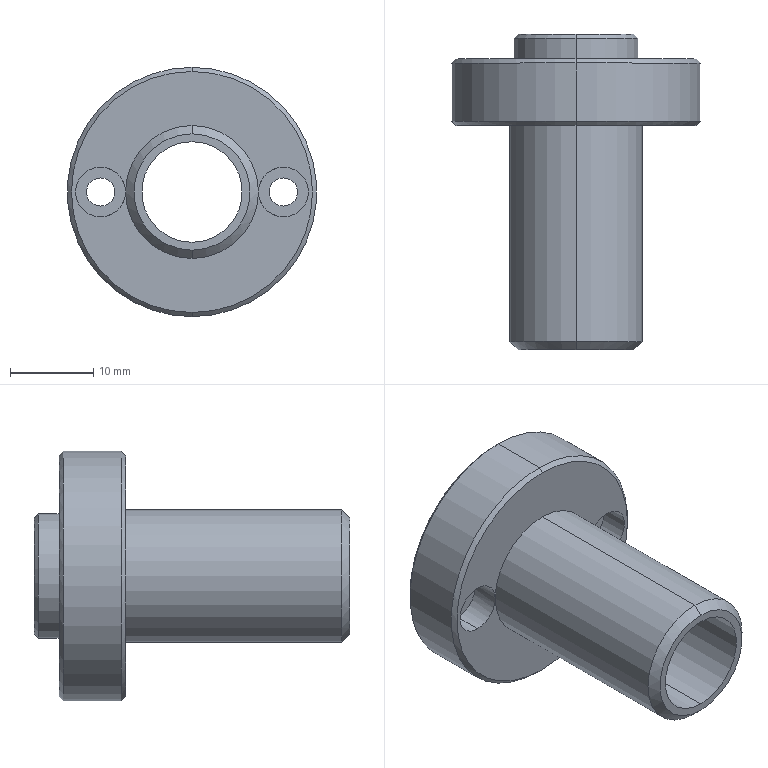Component | SolidWorks | GbgbLowerMagnetGuideTubeF8-1 | 1 solid | 30 faces | box 30 x 38 x 30 mm | volume 6915 mm3 | cylinder 16 | cone 8 | plane 6 | commonest cylinder face diameters 6 x4 3.4 x4 15 x2 30 x2 16 x2 12.1 x2
build123d program:
from build123d import *

# Parameters (mm, degrees)
CHAMFER1_SIZE                                        = 1
HOLE_SIZE_ACCORDING_TO_THE_TYPE_OF_HEX_S_D           = 3.4
HOLE_SIZE_ACCORDING_TO_THE_TYPE_OF_HEX_S_CBORE_D     = 6
HOLE_SIZE_ACCORDING_TO_THE_TYPE_OF_HEX_S_CBORE_DEPTH = 3.4
CHAMFER2_SIZE                                        = 0.5


with BuildPart() as part:
    # Sketch1 → Revolve1 (revolve)
    with BuildSketch(Plane.XY, mode=Mode.PRIVATE) as revolve1_sk:
        Polygon((-6.05, 38), (-6.05, 0), (-8, 0), (-8, 27), (-15, 27), (-15, 35), (-7.5, 35), (-7.5, 38), align=None)
    revolve(revolve1_sk.sketch.rotate(Axis((0, 48.525, 0), (0, -1, 0)), 270), axis=Axis((0, 48.525, 0), (0, -1, 0)))

    # Chamfer1
    chamfer1_edges = [part.edges().sort_by_distance(p)[0] for p in [
        (0, 0, -8),
    ]]
    chamfer(chamfer1_edges, length=CHAMFER1_SIZE)

    # Hole Size according to the type of hex s (through all)
    with Locations(Plane(origin=(0, 27, 0), x_dir=(-1, 0, 0), z_dir=(0, -1, 0))):
        with Locations((11, 0), (-11, 0)):
            CounterBoreHole(HOLE_SIZE_ACCORDING_TO_THE_TYPE_OF_HEX_S_D / 2, HOLE_SIZE_ACCORDING_TO_THE_TYPE_OF_HEX_S_CBORE_D / 2, HOLE_SIZE_ACCORDING_TO_THE_TYPE_OF_HEX_S_CBORE_DEPTH)

    # Chamfer2
    chamfer2_edges = [part.edges().sort_by_distance(p)[0] for p in [
        (0, 38, -7.5),
        (0, 35, -15),
        (0, 27, -15),
    ]]
    chamfer(chamfer2_edges, length=CHAMFER2_SIZE)


solid = part.part

# Placed as in the assembly
solid = solid.moved(Location((80.446, 337.44, 430.232), (0, 0, 0)))
STEP:
#1=CARTESIAN_POINT('',(3.167,14.781,17.214));
#2=VERTEX_POINT('',#1);
#3=CARTESIAN_POINT('',(3.167,14.781,16.663));
#4=VERTEX_POINT('',#3);
#5=CARTESIAN_POINT('',(3.167,14.781,16.938));
#6=DIRECTION('',(0.,1.,0.));
#7=DIRECTION('',(0.,0.,1.));
#8=AXIS2_PLACEMENT_3D('',#5,#6,#7);
#9=CIRCLE('',#8,0.2756);
#10=EDGE_CURVE('',#2,#4,#9,.T.);
#11=ORIENTED_EDGE('',*,*,#10,.F.);
#12=CARTESIAN_POINT('',(3.167,14.761,17.234));
#13=VERTEX_POINT('',#12);
#14=CARTESIAN_POINT('',(3.167,14.781,17.214));
#15=DIRECTION('',(0.,-0.7071,0.7071));
#16=VECTOR('',#15,39.37);
#17=LINE('',#14,#16);
#18=EDGE_CURVE('',#2,#13,#17,.T.);
#19=ORIENTED_EDGE('',*,*,#18,.T.);
#20=CARTESIAN_POINT('',(3.167,14.761,16.643));
#21=VERTEX_POINT('',#20);
#22=CARTESIAN_POINT('',(3.167,14.761,16.938));
#23=DIRECTION('',(0.,-1.,0.));
#24=DIRECTION('',(0.,0.,1.));
#25=AXIS2_PLACEMENT_3D('',#22,#23,#24);
#26=CIRCLE('',#25,0.2953);
#27=EDGE_CURVE('',#21,#13,#26,.T.);
#28=ORIENTED_EDGE('',*,*,#27,.F.);
#29=CARTESIAN_POINT('',(3.167,14.781,16.663));
#30=DIRECTION('',(0.,-0.7071,-0.7071));
#31=VECTOR('',#30,39.37);
#32=LINE('',#29,#31);
#33=EDGE_CURVE('',#4,#21,#32,.T.);
#34=ORIENTED_EDGE('',*,*,#33,.F.);
#35=EDGE_LOOP('',(#11,#19,#28,#34));
#36=FACE_OUTER_BOUND('',#35,.T.);
#37=CARTESIAN_POINT('',(3.167,14.781,16.938));
#38=DIRECTION('',(0.,-1.,0.));
#39=DIRECTION('',(0.,0.,-1.));
#40=AXIS2_PLACEMENT_3D('',#37,#38,#39);
#41=CONICAL_SURFACE('',#40,0.2756,0.7854);
#42=ADVANCED_FACE('',(#36),#41,.T.);
#43=CARTESIAN_POINT('',(3.167,14.348,16.367));
#44=VERTEX_POINT('',#43);
#45=CARTESIAN_POINT('',(3.167,14.348,17.509));
#46=VERTEX_POINT('',#45);
#47=CARTESIAN_POINT('',(3.167,14.348,16.938));
#48=DIRECTION('',(0.,-1.,0.));
#49=DIRECTION('',(0.,0.,-1.));
#50=AXIS2_PLACEMENT_3D('',#47,#48,#49);
#51=CIRCLE('',#50,0.5709);
#52=EDGE_CURVE('',#44,#46,#51,.T.);
#53=ORIENTED_EDGE('',*,*,#52,.F.);
#54=CARTESIAN_POINT('',(3.167,14.368,16.348));
#55=VERTEX_POINT('',#54);
#56=CARTESIAN_POINT('',(3.167,14.368,16.348));
#57=DIRECTION('',(0.,0.7071,-0.7071));
#58=VECTOR('',#57,39.37);
#59=LINE('',#56,#58);
#60=EDGE_CURVE('',#44,#55,#59,.T.);
#61=ORIENTED_EDGE('',*,*,#60,.T.);
#62=CARTESIAN_POINT('',(3.167,14.368,17.529));
#63=VERTEX_POINT('',#62);
#64=CARTESIAN_POINT('',(3.167,14.368,16.938));
#65=DIRECTION('',(0.,1.,0.));
#66=DIRECTION('',(0.,0.,-1.));
#67=AXIS2_PLACEMENT_3D('',#64,#65,#66);
#68=CIRCLE('',#67,0.5906);
#69=EDGE_CURVE('',#63,#55,#68,.T.);
#70=ORIENTED_EDGE('',*,*,#69,.F.);
#71=CARTESIAN_POINT('',(3.167,14.368,17.529));
#72=DIRECTION('',(0.,0.7071,0.7071));
#73=VECTOR('',#72,39.37);
#74=LINE('',#71,#73);
#75=EDGE_CURVE('',#46,#63,#74,.T.);
#76=ORIENTED_EDGE('',*,*,#75,.F.);
#77=EDGE_LOOP('',(#53,#61,#70,#76));
#78=FACE_OUTER_BOUND('',#77,.T.);
#79=CARTESIAN_POINT('',(3.167,14.368,16.938));
#80=DIRECTION('',(0.,1.,0.));
#81=DIRECTION('',(0.,0.,1.));
#82=AXIS2_PLACEMENT_3D('',#79,#80,#81);
#83=CONICAL_SURFACE('',#82,0.5906,0.7854);
#84=ADVANCED_FACE('',(#78),#83,.T.);
#85=CARTESIAN_POINT('',(3.167,14.663,17.509));
#86=VERTEX_POINT('',#85);
#87=CARTESIAN_POINT('',(3.167,14.663,16.367));
#88=VERTEX_POINT('',#87);
#89=CARTESIAN_POINT('',(3.167,14.663,16.938));
#90=DIRECTION('',(0.,1.,0.));
#91=DIRECTION('',(0.,0.,1.));
#92=AXIS2_PLACEMENT_3D('',#89,#90,#91);
#93=CIRCLE('',#92,0.5709);
#94=EDGE_CURVE('',#86,#88,#93,.T.);
#95=ORIENTED_EDGE('',*,*,#94,.F.);
#96=CARTESIAN_POINT('',(3.167,14.643,17.529));
#97=VERTEX_POINT('',#96);
#98=CARTESIAN_POINT('',(3.167,14.663,17.509));
#99=DIRECTION('',(0.,-0.7071,0.7071));
#100=VECTOR('',#99,39.37);
#101=LINE('',#98,#100);
#102=EDGE_CURVE('',#86,#97,#101,.T.);
#103=ORIENTED_EDGE('',*,*,#102,.T.);
#104=CARTESIAN_POINT('',(3.167,14.643,16.348));
#105=VERTEX_POINT('',#104);
#106=CARTESIAN_POINT('',(3.167,14.643,16.938));
#107=DIRECTION('',(0.,-1.,0.));
#108=DIRECTION('',(0.,0.,1.));
#109=AXIS2_PLACEMENT_3D('',#106,#107,#108);
#110=CIRCLE('',#109,0.5906);
#111=EDGE_CURVE('',#105,#97,#110,.T.);
#112=ORIENTED_EDGE('',*,*,#111,.F.);
#113=CARTESIAN_POINT('',(3.167,14.663,16.367));
#114=DIRECTION('',(0.,-0.7071,-0.7071));
#115=VECTOR('',#114,39.37);
#116=LINE('',#113,#115);
#117=EDGE_CURVE('',#88,#105,#116,.T.);
#118=ORIENTED_EDGE('',*,*,#117,.F.);
#119=EDGE_LOOP('',(#95,#103,#112,#118));
#120=FACE_OUTER_BOUND('',#119,.T.);
#121=CARTESIAN_POINT('',(3.167,14.663,16.938));
#122=DIRECTION('',(0.,-1.,0.));
#123=DIRECTION('',(0.,0.,-1.));
#124=AXIS2_PLACEMENT_3D('',#121,#122,#123);
#125=CONICAL_SURFACE('',#124,0.5709,0.7854);
#126=ADVANCED_FACE('',(#120),#125,.T.);
#127=CARTESIAN_POINT('',(2.734,14.482,17.056));
#128=VERTEX_POINT('',#127);
#129=CARTESIAN_POINT('',(2.734,14.482,16.82));
#130=VERTEX_POINT('',#129);
#131=CARTESIAN_POINT('',(2.734,14.482,16.938));
#132=DIRECTION('',(0.,-1.,0.));
#133=DIRECTION('',(0.,0.,-1.));
#134=AXIS2_PLACEMENT_3D('',#131,#132,#133);
#135=CIRCLE('',#134,0.1181);
#136=EDGE_CURVE('',#128,#130,#135,.T.);
#137=ORIENTED_EDGE('',*,*,#136,.F.);
#138=CARTESIAN_POINT('',(2.734,14.348,17.056));
#139=VERTEX_POINT('',#138);
#140=CARTESIAN_POINT('',(2.734,14.348,17.056));
#141=DIRECTION('',(0.,-1.,0.));
#142=VECTOR('',#141,39.37);
#143=LINE('',#140,#142);
#144=EDGE_CURVE('',#128,#139,#143,.T.);
#145=ORIENTED_EDGE('',*,*,#144,.T.);
#146=CARTESIAN_POINT('',(2.734,14.348,16.82));
#147=VERTEX_POINT('',#146);
#148=CARTESIAN_POINT('',(2.734,14.348,16.938));
#149=DIRECTION('',(0.,-1.,0.));
#150=DIRECTION('',(0.,0.,-1.));
#151=AXIS2_PLACEMENT_3D('',#148,#149,#150);
#152=CIRCLE('',#151,0.1181);
#153=EDGE_CURVE('',#139,#147,#152,.T.);
#154=ORIENTED_EDGE('',*,*,#153,.T.);
#155=CARTESIAN_POINT('',(2.734,14.348,16.82));
#156=DIRECTION('',(0.,-1.,0.));
#157=VECTOR('',#156,39.37);
#158=LINE('',#155,#157);
#159=EDGE_CURVE('',#130,#147,#158,.T.);
#160=ORIENTED_EDGE('',*,*,#159,.F.);
#161=EDGE_LOOP('',(#137,#145,#154,#160));
#162=FACE_OUTER_BOUND('',#161,.T.);
#163=CARTESIAN_POINT('',(2.734,14.348,16.938));
#164=DIRECTION('',(0.,-1.,0.));
#165=DIRECTION('',(0.,0.,-1.));
#166=AXIS2_PLACEMENT_3D('',#163,#164,#165);
#167=CYLINDRICAL_SURFACE('',#166,0.1181);
#168=ADVANCED_FACE('',(#162),#167,.F.);
#169=CARTESIAN_POINT('',(2.734,14.663,16.871));
#170=VERTEX_POINT('',#169);
#171=CARTESIAN_POINT('',(2.734,14.663,17.005));
#172=VERTEX_POINT('',#171);
#173=CARTESIAN_POINT('',(2.734,14.663,16.938));
#174=DIRECTION('',(0.,1.,0.));
#175=DIRECTION('',(0.,0.,1.));
#176=AXIS2_PLACEMENT_3D('',#173,#174,#175);
#177=CIRCLE('',#176,0.06693);
#178=EDGE_CURVE('',#170,#172,#177,.T.);
#179=ORIENTED_EDGE('',*,*,#178,.T.);
#180=CARTESIAN_POINT('',(2.734,14.482,17.005));
#181=VERTEX_POINT('',#180);
#182=CARTESIAN_POINT('',(2.734,14.348,17.005));
#183=DIRECTION('',(0.,-1.,0.));
#184=VECTOR('',#183,39.37);
#185=LINE('',#182,#184);
#186=EDGE_CURVE('',#172,#181,#185,.T.);
#187=ORIENTED_EDGE('',*,*,#186,.T.);
#188=CARTESIAN_POINT('',(2.734,14.482,16.871));
#189=VERTEX_POINT('',#188);
#190=CARTESIAN_POINT('',(2.734,14.482,16.938));
#191=DIRECTION('',(0.,-1.,0.));
#192=DIRECTION('',(0.,0.,-1.));
#193=AXIS2_PLACEMENT_3D('',#190,#191,#192);
#194=CIRCLE('',#193,0.06693);
#195=EDGE_CURVE('',#181,#189,#194,.T.);
#196=ORIENTED_EDGE('',*,*,#195,.T.);
#197=CARTESIAN_POINT('',(2.734,14.348,16.871));
#198=DIRECTION('',(0.,-1.,0.));
#199=VECTOR('',#198,39.37);
#200=LINE('',#197,#199);
#201=EDGE_CURVE('',#170,#189,#200,.T.);
#202=ORIENTED_EDGE('',*,*,#201,.F.);
#203=EDGE_LOOP('',(#179,#187,#196,#202));
#204=FACE_OUTER_BOUND('',#203,.T.);
#205=CARTESIAN_POINT('',(2.734,14.348,16.938));
#206=DIRECTION('',(0.,-1.,0.));
#207=DIRECTION('',(0.,0.,-1.));
#208=AXIS2_PLACEMENT_3D('',#205,#206,#207);
#209=CYLINDRICAL_SURFACE('',#208,0.06693);
#210=ADVANCED_FACE('',(#204),#209,.F.);
#211=CARTESIAN_POINT('',(3.6,14.482,17.056));
#212=VERTEX_POINT('',#211);
#213=CARTESIAN_POINT('',(3.6,14.482,16.82));
#214=VERTEX_POINT('',#213);
#215=CARTESIAN_POINT('',(3.6,14.482,16.938));
#216=DIRECTION('',(0.,-1.,0.));
#217=DIRECTION('',(0.,0.,-1.));
#218=AXIS2_PLACEMENT_3D('',#215,#216,#217);
#219=CIRCLE('',#218,0.1181);
#220=EDGE_CURVE('',#212,#214,#219,.T.);
#221=ORIENTED_EDGE('',*,*,#220,.F.);
#222=CARTESIAN_POINT('',(3.6,14.348,17.056));
#223=VERTEX_POINT('',#222);
#224=CARTESIAN_POINT('',(3.6,14.348,17.056));
#225=DIRECTION('',(0.,-1.,0.));
#226=VECTOR('',#225,39.37);
#227=LINE('',#224,#226);
#228=EDGE_CURVE('',#212,#223,#227,.T.);
#229=ORIENTED_EDGE('',*,*,#228,.T.);
#230=CARTESIAN_POINT('',(3.482,14.348,16.938));
#231=VERTEX_POINT('',#230);
#232=CARTESIAN_POINT('',(3.6,14.348,16.938));
#233=DIRECTION('',(0.,-1.,0.));
#234=DIRECTION('',(0.,0.,-1.));
#235=AXIS2_PLACEMENT_3D('',#232,#233,#234);
#236=CIRCLE('',#235,0.1181);
#237=EDGE_CURVE('',#223,#231,#236,.T.);
#238=ORIENTED_EDGE('',*,*,#237,.T.);
#239=CARTESIAN_POINT('',(3.6,14.348,16.82));
#240=VERTEX_POINT('',#239);
#241=CARTESIAN_POINT('',(3.6,14.348,16.938));
#242=DIRECTION('',(0.,-1.,0.));
#243=DIRECTION('',(0.,0.,-1.));
#244=AXIS2_PLACEMENT_3D('',#241,#242,#243);
#245=CIRCLE('',#244,0.1181);
#246=EDGE_CURVE('',#231,#240,#245,.T.);
#247=ORIENTED_EDGE('',*,*,#246,.T.);
#248=CARTESIAN_POINT('',(3.6,14.348,16.82));
#249=DIRECTION('',(0.,-1.,0.));
#250=VECTOR('',#249,39.37);
#251=LINE('',#248,#250);
#252=EDGE_CURVE('',#214,#240,#251,.T.);
#253=ORIENTED_EDGE('',*,*,#252,.F.);
#254=EDGE_LOOP('',(#221,#229,#238,#247,#253));
#255=FACE_OUTER_BOUND('',#254,.T.);
#256=CARTESIAN_POINT('',(3.6,14.348,16.938));
#257=DIRECTION('',(0.,-1.,0.));
#258=DIRECTION('',(0.,0.,-1.));
#259=AXIS2_PLACEMENT_3D('',#256,#257,#258);
#260=CYLINDRICAL_SURFACE('',#259,0.1181);
#261=ADVANCED_FACE('',(#255),#260,.F.);
#262=CARTESIAN_POINT('',(3.6,14.663,16.871));
#263=VERTEX_POINT('',#262);
#264=CARTESIAN_POINT('',(3.6,14.663,17.005));
#265=VERTEX_POINT('',#264);
#266=CARTESIAN_POINT('',(3.6,14.663,16.938));
#267=DIRECTION('',(0.,1.,0.));
#268=DIRECTION('',(0.,0.,1.));
#269=AXIS2_PLACEMENT_3D('',#266,#267,#268);
#270=CIRCLE('',#269,0.06693);
#271=EDGE_CURVE('',#263,#265,#270,.T.);
#272=ORIENTED_EDGE('',*,*,#271,.T.);
#273=CARTESIAN_POINT('',(3.6,14.482,17.005));
#274=VERTEX_POINT('',#273);
#275=CARTESIAN_POINT('',(3.6,14.348,17.005));
#276=DIRECTION('',(0.,-1.,0.));
#277=VECTOR('',#276,39.37);
#278=LINE('',#275,#277);
#279=EDGE_CURVE('',#265,#274,#278,.T.);
#280=ORIENTED_EDGE('',*,*,#279,.T.);
#281=CARTESIAN_POINT('',(3.6,14.482,16.871));
#282=VERTEX_POINT('',#281);
#283=CARTESIAN_POINT('',(3.6,14.482,16.938));
#284=DIRECTION('',(0.,-1.,0.));
#285=DIRECTION('',(0.,0.,-1.));
#286=AXIS2_PLACEMENT_3D('',#283,#284,#285);
#287=CIRCLE('',#286,0.06693);
#288=EDGE_CURVE('',#274,#282,#287,.T.);
#289=ORIENTED_EDGE('',*,*,#288,.T.);
#290=CARTESIAN_POINT('',(3.6,14.348,16.871));
#291=DIRECTION('',(0.,-1.,0.));
#292=VECTOR('',#291,39.37);
#293=LINE('',#290,#292);
#294=EDGE_CURVE('',#263,#282,#293,.T.);
#295=ORIENTED_EDGE('',*,*,#294,.F.);
#296=EDGE_LOOP('',(#272,#280,#289,#295));
#297=FACE_OUTER_BOUND('',#296,.T.);
#298=CARTESIAN_POINT('',(3.6,14.348,16.938));
#299=DIRECTION('',(0.,-1.,0.));
#300=DIRECTION('',(0.,0.,-1.));
#301=AXIS2_PLACEMENT_3D('',#298,#299,#300);
#302=CYLINDRICAL_SURFACE('',#301,0.06693);
#303=ADVANCED_FACE('',(#297),#302,.F.);
#304=CARTESIAN_POINT('',(3.167,13.285,16.663));
#305=VERTEX_POINT('',#304);
#306=CARTESIAN_POINT('',(3.167,13.285,17.214));
#307=VERTEX_POINT('',#306);
#308=CARTESIAN_POINT('',(3.167,13.285,16.938));
#309=DIRECTION('',(0.,-1.,0.));
#310=DIRECTION('',(0.,0.,-1.));
#311=AXIS2_PLACEMENT_3D('',#308,#309,#310);
#312=CIRCLE('',#311,0.2756);
#313=EDGE_CURVE('',#305,#307,#312,.T.);
#314=ORIENTED_EDGE('',*,*,#313,.F.);
#315=CARTESIAN_POINT('',(3.167,13.324,16.623));
#316=VERTEX_POINT('',#315);
#317=CARTESIAN_POINT('',(3.167,13.324,16.623));
#318=DIRECTION('',(0.,0.7071,-0.7071));
#319=VECTOR('',#318,39.37);
#320=LINE('',#317,#319);
#321=EDGE_CURVE('',#305,#316,#320,.T.);
#322=ORIENTED_EDGE('',*,*,#321,.T.);
#323=CARTESIAN_POINT('',(3.167,13.324,17.253));
#324=VERTEX_POINT('',#323);
#325=CARTESIAN_POINT('',(3.167,13.324,16.938));
#326=DIRECTION('',(0.,1.,0.));
#327=DIRECTION('',(0.,0.,-1.));
#328=AXIS2_PLACEMENT_3D('',#325,#326,#327);
#329=CIRCLE('',#328,0.315);
#330=EDGE_CURVE('',#324,#316,#329,.T.);
#331=ORIENTED_EDGE('',*,*,#330,.F.);
#332=CARTESIAN_POINT('',(3.167,13.324,17.253));
#333=DIRECTION('',(0.,0.7071,0.7071));
#334=VECTOR('',#333,39.37);
#335=LINE('',#332,#334);
#336=EDGE_CURVE('',#307,#324,#335,.T.);
#337=ORIENTED_EDGE('',*,*,#336,.F.);
#338=EDGE_LOOP('',(#314,#322,#331,#337));
#339=FACE_OUTER_BOUND('',#338,.T.);
#340=CARTESIAN_POINT('',(3.167,13.324,16.938));
#341=DIRECTION('',(0.,1.,0.));
#342=DIRECTION('',(0.,0.,1.));
#343=AXIS2_PLACEMENT_3D('',#340,#341,#342);
#344=CONICAL_SURFACE('',#343,0.315,0.7854);
#345=ADVANCED_FACE('',(#339),#344,.T.);
#346=CARTESIAN_POINT('',(3.167,14.663,17.234));
#347=VERTEX_POINT('',#346);
#348=CARTESIAN_POINT('',(3.167,14.663,16.643));
#349=VERTEX_POINT('',#348);
#350=CARTESIAN_POINT('',(3.167,14.663,16.938));
#351=DIRECTION('',(0.,1.,0.));
#352=DIRECTION('',(0.,0.,1.));
#353=AXIS2_PLACEMENT_3D('',#350,#351,#352);
#354=CIRCLE('',#353,0.2953);
#355=EDGE_CURVE('',#347,#349,#354,.T.);
#356=ORIENTED_EDGE('',*,*,#355,.T.);
#357=CARTESIAN_POINT('',(3.167,15.195,16.643));
#358=DIRECTION('',(0.,1.,0.));
#359=VECTOR('',#358,39.37);
#360=LINE('',#357,#359);
#361=EDGE_CURVE('',#349,#21,#360,.T.);
#362=ORIENTED_EDGE('',*,*,#361,.T.);
#363=ORIENTED_EDGE('',*,*,#27,.T.);
#364=CARTESIAN_POINT('',(3.167,15.195,17.234));
#365=DIRECTION('',(0.,1.,0.));
#366=VECTOR('',#365,39.37);
#367=LINE('',#364,#366);
#368=EDGE_CURVE('',#347,#13,#367,.T.);
#369=ORIENTED_EDGE('',*,*,#368,.F.);
#370=EDGE_LOOP('',(#356,#362,#363,#369));
#371=FACE_OUTER_BOUND('',#370,.T.);
#372=CARTESIAN_POINT('',(3.167,15.195,16.938));
#373=DIRECTION('',(0.,1.,0.));
#374=DIRECTION('',(0.,0.,1.));
#375=AXIS2_PLACEMENT_3D('',#372,#373,#374);
#376=CYLINDRICAL_SURFACE('',#375,0.2953);
#377=ADVANCED_FACE('',(#371),#376,.T.);
#378=ORIENTED_EDGE('',*,*,#69,.T.);
#379=CARTESIAN_POINT('',(3.167,15.195,16.348));
#380=DIRECTION('',(0.,1.,0.));
#381=VECTOR('',#380,39.37);
#382=LINE('',#379,#381);
#383=EDGE_CURVE('',#55,#105,#382,.T.);
#384=ORIENTED_EDGE('',*,*,#383,.T.);
#385=ORIENTED_EDGE('',*,*,#111,.T.);
#386=CARTESIAN_POINT('',(3.167,15.195,17.529));
#387=DIRECTION('',(0.,1.,0.));
#388=VECTOR('',#387,39.37);
#389=LINE('',#386,#388);
#390=EDGE_CURVE('',#63,#97,#389,.T.);
#391=ORIENTED_EDGE('',*,*,#390,.F.);
#392=EDGE_LOOP('',(#378,#384,#385,#391));
#393=FACE_OUTER_BOUND('',#392,.T.);
#394=CARTESIAN_POINT('',(3.167,15.195,16.938));
#395=DIRECTION('',(0.,1.,0.));
#396=DIRECTION('',(0.,0.,1.));
#397=AXIS2_PLACEMENT_3D('',#394,#395,#396);
#398=CYLINDRICAL_SURFACE('',#397,0.5906);
#399=ADVANCED_FACE('',(#393),#398,.T.);
#400=ORIENTED_EDGE('',*,*,#330,.T.);
#401=CARTESIAN_POINT('',(3.167,14.348,16.623));
#402=VERTEX_POINT('',#401);
#403=CARTESIAN_POINT('',(3.167,15.195,16.623));
#404=DIRECTION('',(0.,1.,0.));
#405=VECTOR('',#404,39.37);
#406=LINE('',#403,#405);
#407=EDGE_CURVE('',#316,#402,#406,.T.);
#408=ORIENTED_EDGE('',*,*,#407,.T.);
#409=CARTESIAN_POINT('',(3.167,14.348,16.938));
#410=DIRECTION('',(0.,1.,0.));
#411=DIRECTION('',(0.,0.,1.));
#412=AXIS2_PLACEMENT_3D('',#409,#410,#411);
#413=CIRCLE('',#412,0.315);
#414=EDGE_CURVE('',#231,#402,#413,.T.);
#415=ORIENTED_EDGE('',*,*,#414,.F.);
#416=CARTESIAN_POINT('',(3.167,14.348,17.253));
#417=VERTEX_POINT('',#416);
#418=CARTESIAN_POINT('',(3.167,14.348,16.938));
#419=DIRECTION('',(0.,1.,0.));
#420=DIRECTION('',(0.,0.,1.));
#421=AXIS2_PLACEMENT_3D('',#418,#419,#420);
#422=CIRCLE('',#421,0.315);
#423=EDGE_CURVE('',#417,#231,#422,.T.);
#424=ORIENTED_EDGE('',*,*,#423,.F.);
#425=CARTESIAN_POINT('',(3.167,15.195,17.253));
#426=DIRECTION('',(0.,1.,0.));
#427=VECTOR('',#426,39.37);
#428=LINE('',#425,#427);
#429=EDGE_CURVE('',#324,#417,#428,.T.);
#430=ORIENTED_EDGE('',*,*,#429,.F.);
#431=EDGE_LOOP('',(#400,#408,#415,#424,#430));
#432=FACE_OUTER_BOUND('',#431,.T.);
#433=CARTESIAN_POINT('',(3.167,15.195,16.938));
#434=DIRECTION('',(0.,1.,0.));
#435=DIRECTION('',(0.,0.,1.));
#436=AXIS2_PLACEMENT_3D('',#433,#434,#435);
#437=CYLINDRICAL_SURFACE('',#436,0.315);
#438=ADVANCED_FACE('',(#432),#437,.T.);
#439=CARTESIAN_POINT('',(3.167,13.285,16.7));
#440=VERTEX_POINT('',#439);
#441=CARTESIAN_POINT('',(3.167,13.285,17.176));
#442=VERTEX_POINT('',#441);
#443=CARTESIAN_POINT('',(3.167,13.285,16.938));
#444=DIRECTION('',(0.,1.,0.));
#445=DIRECTION('',(0.,0.,1.));
#446=AXIS2_PLACEMENT_3D('',#443,#444,#445);
#447=CIRCLE('',#446,0.2382);
#448=EDGE_CURVE('',#440,#442,#447,.T.);
#449=ORIENTED_EDGE('',*,*,#448,.F.);
#450=CARTESIAN_POINT('',(3.167,14.781,16.7));
#451=VERTEX_POINT('',#450);
#452=CARTESIAN_POINT('',(3.167,15.195,16.7));
#453=DIRECTION('',(0.,1.,0.));
#454=VECTOR('',#453,39.37);
#455=LINE('',#452,#454);
#456=EDGE_CURVE('',#440,#451,#455,.T.);
#457=ORIENTED_EDGE('',*,*,#456,.T.);
#458=CARTESIAN_POINT('',(3.167,14.781,17.176));
#459=VERTEX_POINT('',#458);
#460=CARTESIAN_POINT('',(3.167,14.781,16.938));
#461=DIRECTION('',(0.,1.,0.));
#462=DIRECTION('',(0.,0.,1.));
#463=AXIS2_PLACEMENT_3D('',#460,#461,#462);
#464=CIRCLE('',#463,0.2382);
#465=EDGE_CURVE('',#451,#459,#464,.T.);
#466=ORIENTED_EDGE('',*,*,#465,.T.);
#467=CARTESIAN_POINT('',(3.167,15.195,17.176));
#468=DIRECTION('',(0.,1.,0.));
#469=VECTOR('',#468,39.37);
#470=LINE('',#467,#469);
#471=EDGE_CURVE('',#442,#459,#470,.T.);
#472=ORIENTED_EDGE('',*,*,#471,.F.);
#473=EDGE_LOOP('',(#449,#457,#466,#472));
#474=FACE_OUTER_BOUND('',#473,.T.);
#475=CARTESIAN_POINT('',(3.167,15.195,16.938));
#476=DIRECTION('',(0.,1.,0.));
#477=DIRECTION('',(0.,0.,1.));
#478=AXIS2_PLACEMENT_3D('',#475,#476,#477);
#479=CYLINDRICAL_SURFACE('',#478,0.2382);
#480=ADVANCED_FACE('',(#474),#479,.F.);
#481=CARTESIAN_POINT('',(3.167,14.781,16.938));
#482=DIRECTION('',(0.,1.,0.));
#483=DIRECTION('',(0.,0.,1.));
#484=AXIS2_PLACEMENT_3D('',#481,#482,#483);
#485=CIRCLE('',#484,0.2756);
#486=EDGE_CURVE('',#4,#2,#485,.T.);
#487=ORIENTED_EDGE('',*,*,#486,.T.);
#488=ORIENTED_EDGE('',*,*,#10,.T.);
#489=EDGE_LOOP('',(#487,#488));
#490=FACE_OUTER_BOUND('',#489,.T.);
#491=CARTESIAN_POINT('',(3.167,14.781,16.938));
#492=DIRECTION('',(0.,1.,0.));
#493=DIRECTION('',(0.,0.,1.));
#494=AXIS2_PLACEMENT_3D('',#491,#492,#493);
#495=CIRCLE('',#494,0.2382);
#496=EDGE_CURVE('',#459,#451,#495,.T.);
#497=ORIENTED_EDGE('',*,*,#496,.F.);
#498=ORIENTED_EDGE('',*,*,#465,.F.);
#499=EDGE_LOOP('',(#497,#498));
#500=FACE_BOUND('',#499,.T.);
#501=CARTESIAN_POINT('',(2.872,14.781,16.938));
#502=DIRECTION('',(0.,1.,0.));
#503=DIRECTION('',(0.,0.,1.));
#504=AXIS2_PLACEMENT_3D('',#501,#502,#503);
#505=PLANE('',#504);
#506=ADVANCED_FACE('',(#490,#500),#505,.T.);
#507=ORIENTED_EDGE('',*,*,#456,.F.);
#508=CARTESIAN_POINT('',(3.167,13.285,16.938));
#509=DIRECTION('',(0.,1.,0.));
#510=DIRECTION('',(0.,0.,1.));
#511=AXIS2_PLACEMENT_3D('',#508,#509,#510);
#512=CIRCLE('',#511,0.2382);
#513=EDGE_CURVE('',#442,#440,#512,.T.);
#514=ORIENTED_EDGE('',*,*,#513,.F.);
#515=ORIENTED_EDGE('',*,*,#471,.T.);
#516=ORIENTED_EDGE('',*,*,#496,.T.);
#517=EDGE_LOOP('',(#507,#514,#515,#516));
#518=FACE_OUTER_BOUND('',#517,.T.);
#519=CARTESIAN_POINT('',(3.167,15.195,16.938));
#520=DIRECTION('',(0.,1.,0.));
#521=DIRECTION('',(0.,0.,1.));
#522=AXIS2_PLACEMENT_3D('',#519,#520,#521);
#523=CYLINDRICAL_SURFACE('',#522,0.2382);
#524=ADVANCED_FACE('',(#518),#523,.F.);
#525=CARTESIAN_POINT('',(3.167,13.285,16.938));
#526=DIRECTION('',(0.,-1.,0.));
#527=DIRECTION('',(0.,0.,-1.));
#528=AXIS2_PLACEMENT_3D('',#525,#526,#527);
#529=CIRCLE('',#528,0.2756);
#530=EDGE_CURVE('',#307,#305,#529,.T.);
#531=ORIENTED_EDGE('',*,*,#530,.T.);
#532=ORIENTED_EDGE('',*,*,#313,.T.);
#533=EDGE_LOOP('',(#531,#532));
#534=FACE_OUTER_BOUND('',#533,.T.);
#535=ORIENTED_EDGE('',*,*,#513,.T.);
#536=ORIENTED_EDGE('',*,*,#448,.T.);
#537=EDGE_LOOP('',(#535,#536));
#538=FACE_BOUND('',#537,.T.);
#539=CARTESIAN_POINT('',(2.929,13.285,16.938));
#540=DIRECTION('',(0.,-1.,0.));
#541=DIRECTION('',(0.,0.,-1.));
#542=AXIS2_PLACEMENT_3D('',#539,#540,#541);
#543=PLANE('',#542);
#544=ADVANCED_FACE('',(#534,#538),#543,.T.);
#545=ORIENTED_EDGE('',*,*,#407,.F.);
#546=CARTESIAN_POINT('',(3.167,13.324,16.938));
#547=DIRECTION('',(0.,1.,0.));
#548=DIRECTION('',(0.,0.,-1.));
#549=AXIS2_PLACEMENT_3D('',#546,#547,#548);
#550=CIRCLE('',#549,0.315);
#551=EDGE_CURVE('',#316,#324,#550,.T.);
#552=ORIENTED_EDGE('',*,*,#551,.T.);
#553=ORIENTED_EDGE('',*,*,#429,.T.);
#554=CARTESIAN_POINT('',(2.852,14.348,16.938));
#555=VERTEX_POINT('',#554);
#556=CARTESIAN_POINT('',(3.167,14.348,16.938));
#557=DIRECTION('',(0.,1.,0.));
#558=DIRECTION('',(0.,0.,1.));
#559=AXIS2_PLACEMENT_3D('',#556,#557,#558);
#560=CIRCLE('',#559,0.315);
#561=EDGE_CURVE('',#555,#417,#560,.T.);
#562=ORIENTED_EDGE('',*,*,#561,.F.);
#563=CARTESIAN_POINT('',(3.167,14.348,16.938));
#564=DIRECTION('',(0.,1.,0.));
#565=DIRECTION('',(0.,0.,1.));
#566=AXIS2_PLACEMENT_3D('',#563,#564,#565);
#567=CIRCLE('',#566,0.315);
#568=EDGE_CURVE('',#402,#555,#567,.T.);
#569=ORIENTED_EDGE('',*,*,#568,.F.);
#570=EDGE_LOOP('',(#545,#552,#553,#562,#569));
#571=FACE_OUTER_BOUND('',#570,.T.);
#572=CARTESIAN_POINT('',(3.167,15.195,16.938));
#573=DIRECTION('',(0.,1.,0.));
#574=DIRECTION('',(0.,0.,1.));
#575=AXIS2_PLACEMENT_3D('',#572,#573,#574);
#576=CYLINDRICAL_SURFACE('',#575,0.315);
#577=ADVANCED_FACE('',(#571),#576,.T.);
#578=CARTESIAN_POINT('',(3.167,14.348,16.938));
#579=DIRECTION('',(0.,-1.,0.));
#580=DIRECTION('',(0.,0.,-1.));
#581=AXIS2_PLACEMENT_3D('',#578,#579,#580);
#582=CIRCLE('',#581,0.5709);
#583=EDGE_CURVE('',#46,#44,#582,.T.);
#584=ORIENTED_EDGE('',*,*,#583,.T.);
#585=ORIENTED_EDGE('',*,*,#52,.T.);
#586=EDGE_LOOP('',(#584,#585));
#587=FACE_OUTER_BOUND('',#586,.T.);
#588=ORIENTED_EDGE('',*,*,#414,.T.);
#589=ORIENTED_EDGE('',*,*,#568,.T.);
#590=CARTESIAN_POINT('',(2.734,14.348,16.938));
#591=DIRECTION('',(0.,-1.,0.));
#592=DIRECTION('',(0.,0.,-1.));
#593=AXIS2_PLACEMENT_3D('',#590,#591,#592);
#594=CIRCLE('',#593,0.1181);
#595=EDGE_CURVE('',#147,#555,#594,.T.);
#596=ORIENTED_EDGE('',*,*,#595,.F.);
#597=ORIENTED_EDGE('',*,*,#153,.F.);
#598=CARTESIAN_POINT('',(2.734,14.348,16.938));
#599=DIRECTION('',(0.,-1.,0.));
#600=DIRECTION('',(0.,0.,-1.));
#601=AXIS2_PLACEMENT_3D('',#598,#599,#600);
#602=CIRCLE('',#601,0.1181);
#603=EDGE_CURVE('',#555,#139,#602,.T.);
#604=ORIENTED_EDGE('',*,*,#603,.F.);
#605=ORIENTED_EDGE('',*,*,#561,.T.);
#606=ORIENTED_EDGE('',*,*,#423,.T.);
#607=ORIENTED_EDGE('',*,*,#237,.F.);
#608=CARTESIAN_POINT('',(3.6,14.348,16.938));
#609=DIRECTION('',(0.,-1.,0.));
#610=DIRECTION('',(0.,0.,-1.));
#611=AXIS2_PLACEMENT_3D('',#608,#609,#610);
#612=CIRCLE('',#611,0.1181);
#613=EDGE_CURVE('',#240,#223,#612,.T.);
#614=ORIENTED_EDGE('',*,*,#613,.F.);
#615=ORIENTED_EDGE('',*,*,#246,.F.);
#616=EDGE_LOOP('',(#588,#589,#596,#597,#604,#605,#606,#607,#614,#615));
#617=FACE_BOUND('',#616,.T.);
#618=CARTESIAN_POINT('',(2.852,14.348,16.938));
#619=DIRECTION('',(0.,-1.,0.));
#620=DIRECTION('',(0.,0.,-1.));
#621=AXIS2_PLACEMENT_3D('',#618,#619,#620);
#622=PLANE('',#621);
#623=ADVANCED_FACE('',(#587,#617),#622,.T.);
#624=ORIENTED_EDGE('',*,*,#383,.F.);
#625=CARTESIAN_POINT('',(3.167,14.368,16.938));
#626=DIRECTION('',(0.,1.,0.));
#627=DIRECTION('',(0.,0.,-1.));
#628=AXIS2_PLACEMENT_3D('',#625,#626,#627);
#629=CIRCLE('',#628,0.5906);
#630=EDGE_CURVE('',#55,#63,#629,.T.);
#631=ORIENTED_EDGE('',*,*,#630,.T.);
#632=ORIENTED_EDGE('',*,*,#390,.T.);
#633=CARTESIAN_POINT('',(3.167,14.643,16.938));
#634=DIRECTION('',(0.,-1.,0.));
#635=DIRECTION('',(0.,0.,1.));
#636=AXIS2_PLACEMENT_3D('',#633,#634,#635);
#637=CIRCLE('',#636,0.5906);
#638=EDGE_CURVE('',#97,#105,#637,.T.);
#639=ORIENTED_EDGE('',*,*,#638,.T.);
#640=EDGE_LOOP('',(#624,#631,#632,#639));
#641=FACE_OUTER_BOUND('',#640,.T.);
#642=CARTESIAN_POINT('',(3.167,15.195,16.938));
#643=DIRECTION('',(0.,1.,0.));
#644=DIRECTION('',(0.,0.,1.));
#645=AXIS2_PLACEMENT_3D('',#642,#643,#644);
#646=CYLINDRICAL_SURFACE('',#645,0.5906);
#647=ADVANCED_FACE('',(#641),#646,.T.);
#648=CARTESIAN_POINT('',(3.167,14.663,16.938));
#649=DIRECTION('',(0.,1.,0.));
#650=DIRECTION('',(0.,0.,1.));
#651=AXIS2_PLACEMENT_3D('',#648,#649,#650);
#652=CIRCLE('',#651,0.5709);
#653=EDGE_CURVE('',#88,#86,#652,.T.);
#654=ORIENTED_EDGE('',*,*,#653,.T.);
#655=ORIENTED_EDGE('',*,*,#94,.T.);
#656=EDGE_LOOP('',(#654,#655));
#657=FACE_OUTER_BOUND('',#656,.T.);
#658=ORIENTED_EDGE('',*,*,#178,.F.);
#659=CARTESIAN_POINT('',(2.734,14.663,16.938));
#660=DIRECTION('',(0.,1.,0.));
#661=DIRECTION('',(0.,0.,1.));
#662=AXIS2_PLACEMENT_3D('',#659,#660,#661);
#663=CIRCLE('',#662,0.06693);
#664=EDGE_CURVE('',#172,#170,#663,.T.);
#665=ORIENTED_EDGE('',*,*,#664,.F.);
#666=EDGE_LOOP('',(#658,#665));
#667=FACE_BOUND('',#666,.T.);
#668=ORIENTED_EDGE('',*,*,#271,.F.);
#669=CARTESIAN_POINT('',(3.6,14.663,16.938));
#670=DIRECTION('',(0.,1.,0.));
#671=DIRECTION('',(0.,0.,1.));
#672=AXIS2_PLACEMENT_3D('',#669,#670,#671);
#673=CIRCLE('',#672,0.06693);
#674=EDGE_CURVE('',#265,#263,#673,.T.);
#675=ORIENTED_EDGE('',*,*,#674,.F.);
#676=EDGE_LOOP('',(#668,#675));
#677=FACE_BOUND('',#676,.T.);
#678=ORIENTED_EDGE('',*,*,#355,.F.);
#679=CARTESIAN_POINT('',(3.167,14.663,16.938));
#680=DIRECTION('',(0.,1.,0.));
#681=DIRECTION('',(0.,0.,1.));
#682=AXIS2_PLACEMENT_3D('',#679,#680,#681);
#683=CIRCLE('',#682,0.2953);
#684=EDGE_CURVE('',#349,#347,#683,.T.);
#685=ORIENTED_EDGE('',*,*,#684,.F.);
#686=EDGE_LOOP('',(#678,#685));
#687=FACE_BOUND('',#686,.T.);
#688=CARTESIAN_POINT('',(2.577,14.663,16.938));
#689=DIRECTION('',(0.,1.,0.));
#690=DIRECTION('',(0.,0.,1.));
#691=AXIS2_PLACEMENT_3D('',#688,#689,#690);
#692=PLANE('',#691);
#693=ADVANCED_FACE('',(#657,#667,#677,#687),#692,.T.);
#694=ORIENTED_EDGE('',*,*,#361,.F.);
#695=ORIENTED_EDGE('',*,*,#684,.T.);
#696=ORIENTED_EDGE('',*,*,#368,.T.);
#697=CARTESIAN_POINT('',(3.167,14.761,16.938));
#698=DIRECTION('',(0.,-1.,0.));
#699=DIRECTION('',(0.,0.,1.));
#700=AXIS2_PLACEMENT_3D('',#697,#698,#699);
#701=CIRCLE('',#700,0.2953);
#702=EDGE_CURVE('',#13,#21,#701,.T.);
#703=ORIENTED_EDGE('',*,*,#702,.T.);
#704=EDGE_LOOP('',(#694,#695,#696,#703));
#705=FACE_OUTER_BOUND('',#704,.T.);
#706=CARTESIAN_POINT('',(3.167,15.195,16.938));
#707=DIRECTION('',(0.,1.,0.));
#708=DIRECTION('',(0.,0.,1.));
#709=AXIS2_PLACEMENT_3D('',#706,#707,#708);
#710=CYLINDRICAL_SURFACE('',#709,0.2953);
#711=ADVANCED_FACE('',(#705),#710,.T.);
#712=ORIENTED_EDGE('',*,*,#321,.F.);
#713=ORIENTED_EDGE('',*,*,#530,.F.);
#714=ORIENTED_EDGE('',*,*,#336,.T.);
#715=ORIENTED_EDGE('',*,*,#551,.F.);
#716=EDGE_LOOP('',(#712,#713,#714,#715));
#717=FACE_OUTER_BOUND('',#716,.T.);
#718=CARTESIAN_POINT('',(3.167,13.324,16.938));
#719=DIRECTION('',(0.,1.,0.));
#720=DIRECTION('',(0.,0.,1.));
#721=AXIS2_PLACEMENT_3D('',#718,#719,#720);
#722=CONICAL_SURFACE('',#721,0.315,0.7854);
#723=ADVANCED_FACE('',(#717),#722,.T.);
#724=ORIENTED_EDGE('',*,*,#279,.F.);
#725=ORIENTED_EDGE('',*,*,#674,.T.);
#726=ORIENTED_EDGE('',*,*,#294,.T.);
#727=CARTESIAN_POINT('',(3.6,14.482,16.938));
#728=DIRECTION('',(0.,-1.,0.));
#729=DIRECTION('',(0.,0.,-1.));
#730=AXIS2_PLACEMENT_3D('',#727,#728,#729);
#731=CIRCLE('',#730,0.06693);
#732=EDGE_CURVE('',#282,#274,#731,.T.);
#733=ORIENTED_EDGE('',*,*,#732,.T.);
#734=EDGE_LOOP('',(#724,#725,#726,#733));
#735=FACE_OUTER_BOUND('',#734,.T.);
#736=CARTESIAN_POINT('',(3.6,14.348,16.938));
#737=DIRECTION('',(0.,-1.,0.));
#738=DIRECTION('',(0.,0.,-1.));
#739=AXIS2_PLACEMENT_3D('',#736,#737,#738);
#740=CYLINDRICAL_SURFACE('',#739,0.06693);
#741=ADVANCED_FACE('',(#735),#740,.F.);
#742=ORIENTED_EDGE('',*,*,#732,.F.);
#743=ORIENTED_EDGE('',*,*,#288,.F.);
#744=EDGE_LOOP('',(#742,#743));
#745=FACE_BOUND('',#744,.T.);
#746=CARTESIAN_POINT('',(3.6,14.482,16.938));
#747=DIRECTION('',(0.,-1.,0.));
#748=DIRECTION('',(0.,0.,-1.));
#749=AXIS2_PLACEMENT_3D('',#746,#747,#748);
#750=CIRCLE('',#749,0.1181);
#751=EDGE_CURVE('',#214,#212,#750,.T.);
#752=ORIENTED_EDGE('',*,*,#751,.T.);
#753=ORIENTED_EDGE('',*,*,#220,.T.);
#754=EDGE_LOOP('',(#752,#753));
#755=FACE_OUTER_BOUND('',#754,.T.);
#756=CARTESIAN_POINT('',(3.667,14.482,16.938));
#757=DIRECTION('',(0.,1.,0.));
#758=DIRECTION('',(0.,0.,1.));
#759=AXIS2_PLACEMENT_3D('',#756,#757,#758);
#760=PLANE('',#759);
#761=ADVANCED_FACE('',(#745,#755),#760,.F.);
#762=ORIENTED_EDGE('',*,*,#228,.F.);
#763=ORIENTED_EDGE('',*,*,#751,.F.);
#764=ORIENTED_EDGE('',*,*,#252,.T.);
#765=ORIENTED_EDGE('',*,*,#613,.T.);
#766=EDGE_LOOP('',(#762,#763,#764,#765));
#767=FACE_OUTER_BOUND('',#766,.T.);
#768=CARTESIAN_POINT('',(3.6,14.348,16.938));
#769=DIRECTION('',(0.,-1.,0.));
#770=DIRECTION('',(0.,0.,-1.));
#771=AXIS2_PLACEMENT_3D('',#768,#769,#770);
#772=CYLINDRICAL_SURFACE('',#771,0.1181);
#773=ADVANCED_FACE('',(#767),#772,.F.);
#774=ORIENTED_EDGE('',*,*,#186,.F.);
#775=ORIENTED_EDGE('',*,*,#664,.T.);
#776=ORIENTED_EDGE('',*,*,#201,.T.);
#777=CARTESIAN_POINT('',(2.734,14.482,16.938));
#778=DIRECTION('',(0.,-1.,0.));
#779=DIRECTION('',(0.,0.,-1.));
#780=AXIS2_PLACEMENT_3D('',#777,#778,#779);
#781=CIRCLE('',#780,0.06693);
#782=EDGE_CURVE('',#189,#181,#781,.T.);
#783=ORIENTED_EDGE('',*,*,#782,.T.);
#784=EDGE_LOOP('',(#774,#775,#776,#783));
#785=FACE_OUTER_BOUND('',#784,.T.);
#786=CARTESIAN_POINT('',(2.734,14.348,16.938));
#787=DIRECTION('',(0.,-1.,0.));
#788=DIRECTION('',(0.,0.,-1.));
#789=AXIS2_PLACEMENT_3D('',#786,#787,#788);
#790=CYLINDRICAL_SURFACE('',#789,0.06693);
#791=ADVANCED_FACE('',(#785),#790,.F.);
#792=ORIENTED_EDGE('',*,*,#782,.F.);
#793=ORIENTED_EDGE('',*,*,#195,.F.);
#794=EDGE_LOOP('',(#792,#793));
#795=FACE_BOUND('',#794,.T.);
#796=CARTESIAN_POINT('',(2.734,14.482,16.938));
#797=DIRECTION('',(0.,-1.,0.));
#798=DIRECTION('',(0.,0.,-1.));
#799=AXIS2_PLACEMENT_3D('',#796,#797,#798);
#800=CIRCLE('',#799,0.1181);
#801=EDGE_CURVE('',#130,#128,#800,.T.);
#802=ORIENTED_EDGE('',*,*,#801,.T.);
#803=ORIENTED_EDGE('',*,*,#136,.T.);
#804=EDGE_LOOP('',(#802,#803));
#805=FACE_OUTER_BOUND('',#804,.T.);
#806=CARTESIAN_POINT('',(2.801,14.482,16.938));
#807=DIRECTION('',(0.,1.,0.));
#808=DIRECTION('',(0.,0.,1.));
#809=AXIS2_PLACEMENT_3D('',#806,#807,#808);
#810=PLANE('',#809);
#811=ADVANCED_FACE('',(#795,#805),#810,.F.);
#812=ORIENTED_EDGE('',*,*,#144,.F.);
#813=ORIENTED_EDGE('',*,*,#801,.F.);
#814=ORIENTED_EDGE('',*,*,#159,.T.);
#815=ORIENTED_EDGE('',*,*,#595,.T.);
#816=ORIENTED_EDGE('',*,*,#603,.T.);
#817=EDGE_LOOP('',(#812,#813,#814,#815,#816));
#818=FACE_OUTER_BOUND('',#817,.T.);
#819=CARTESIAN_POINT('',(2.734,14.348,16.938));
#820=DIRECTION('',(0.,-1.,0.));
#821=DIRECTION('',(0.,0.,-1.));
#822=AXIS2_PLACEMENT_3D('',#819,#820,#821);
#823=CYLINDRICAL_SURFACE('',#822,0.1181);
#824=ADVANCED_FACE('',(#818),#823,.F.);
#825=ORIENTED_EDGE('',*,*,#102,.F.);
#826=ORIENTED_EDGE('',*,*,#653,.F.);
#827=ORIENTED_EDGE('',*,*,#117,.T.);
#828=ORIENTED_EDGE('',*,*,#638,.F.);
#829=EDGE_LOOP('',(#825,#826,#827,#828));
#830=FACE_OUTER_BOUND('',#829,.T.);
#831=CARTESIAN_POINT('',(3.167,14.663,16.938));
#832=DIRECTION('',(0.,-1.,0.));
#833=DIRECTION('',(0.,0.,-1.));
#834=AXIS2_PLACEMENT_3D('',#831,#832,#833);
#835=CONICAL_SURFACE('',#834,0.5709,0.7854);
#836=ADVANCED_FACE('',(#830),#835,.T.);
#837=ORIENTED_EDGE('',*,*,#60,.F.);
#838=ORIENTED_EDGE('',*,*,#583,.F.);
#839=ORIENTED_EDGE('',*,*,#75,.T.);
#840=ORIENTED_EDGE('',*,*,#630,.F.);
#841=EDGE_LOOP('',(#837,#838,#839,#840));
#842=FACE_OUTER_BOUND('',#841,.T.);
#843=CARTESIAN_POINT('',(3.167,14.368,16.938));
#844=DIRECTION('',(0.,1.,0.));
#845=DIRECTION('',(0.,0.,1.));
#846=AXIS2_PLACEMENT_3D('',#843,#844,#845);
#847=CONICAL_SURFACE('',#846,0.5906,0.7854);
#848=ADVANCED_FACE('',(#842),#847,.T.);
#849=ORIENTED_EDGE('',*,*,#18,.F.);
#850=ORIENTED_EDGE('',*,*,#486,.F.);
#851=ORIENTED_EDGE('',*,*,#33,.T.);
#852=ORIENTED_EDGE('',*,*,#702,.F.);
#853=EDGE_LOOP('',(#849,#850,#851,#852));
#854=FACE_OUTER_BOUND('',#853,.T.);
#855=CARTESIAN_POINT('',(3.167,14.781,16.938));
#856=DIRECTION('',(0.,-1.,0.));
#857=DIRECTION('',(0.,0.,-1.));
#858=AXIS2_PLACEMENT_3D('',#855,#856,#857);
#859=CONICAL_SURFACE('',#858,0.2756,0.7854);
#860=ADVANCED_FACE('',(#854),#859,.T.);
#861=CLOSED_SHELL('',(#42,#84,#126,#168,#210,#261,#303,#345,#377,#399,#438,#480,#506,#524,#544,#577,#623,#647,#693,#711,#723,#741,#761,#773,#791,#811,#824,#836,#848,#860));
#862=MANIFOLD_SOLID_BREP('',#861);
#863=CARTESIAN_POINT('',(0.,0.,0.));
#864=DIRECTION('',(0.,0.,1.));
#865=DIRECTION('',(1.,0.,0.));
#866=AXIS2_PLACEMENT_3D('',#863,#864,#865);
#867=(LENGTH_UNIT()NAMED_UNIT(*)SI_UNIT($,.METRE.));
#868=LENGTH_MEASURE_WITH_UNIT(LENGTH_MEASURE(0.0254),#867);
#869=DIMENSIONAL_EXPONENTS(1.,0.,0.,0.,0.,0.,0.);
#870=(CONVERSION_BASED_UNIT('',#868)LENGTH_UNIT()NAMED_UNIT(#869));
#871=UNCERTAINTY_MEASURE_WITH_UNIT(LENGTH_MEASURE(0.00001),#870,'','');
#872=(NAMED_UNIT(*)PLANE_ANGLE_UNIT()SI_UNIT($,.RADIAN.));
#873=(NAMED_UNIT(*)SI_UNIT($,.STERADIAN.)SOLID_ANGLE_UNIT());
#874=(GEOMETRIC_REPRESENTATION_CONTEXT(3)GLOBAL_UNCERTAINTY_ASSIGNED_CONTEXT((#871))GLOBAL_UNIT_ASSIGNED_CONTEXT((#870,#872,#873))REPRESENTATION_CONTEXT('',''));
#875=ADVANCED_BREP_SHAPE_REPRESENTATION('',(#862,#866),#874);
#876=COLOUR_RGB('',0.7922,0.8196,0.9333);
#877=FILL_AREA_STYLE_COLOUR('',#876);
#878=FILL_AREA_STYLE('',(#877));
#879=SURFACE_STYLE_FILL_AREA(#878);
#880=SURFACE_SIDE_STYLE('',(#879));
#881=SURFACE_STYLE_USAGE(.BOTH.,#880);
#882=PRESENTATION_STYLE_ASSIGNMENT((#881));
#883=STYLED_ITEM('',(#882),#862);
#884=(LENGTH_UNIT()NAMED_UNIT(*)SI_UNIT($,.METRE.));
#885=LENGTH_MEASURE_WITH_UNIT(LENGTH_MEASURE(0.0254),#884);
#886=DIMENSIONAL_EXPONENTS(1.,0.,0.,0.,0.,0.,0.);
#887=(CONVERSION_BASED_UNIT('',#885)LENGTH_UNIT()NAMED_UNIT(#886));
#888=UNCERTAINTY_MEASURE_WITH_UNIT(LENGTH_MEASURE(0.00001),#887,'','');
#889=(NAMED_UNIT(*)PLANE_ANGLE_UNIT()SI_UNIT($,.RADIAN.));
#890=(NAMED_UNIT(*)SI_UNIT($,.STERADIAN.)SOLID_ANGLE_UNIT());
#891=(GEOMETRIC_REPRESENTATION_CONTEXT(3)GLOBAL_UNCERTAINTY_ASSIGNED_CONTEXT((#888))GLOBAL_UNIT_ASSIGNED_CONTEXT((#887,#889,#890))REPRESENTATION_CONTEXT('',''));
#892=MECHANICAL_DESIGN_GEOMETRIC_PRESENTATION_REPRESENTATION('',(#883),#891);
#893=PRESENTATION_LAYER_ASSIGNMENT('','',(#883));